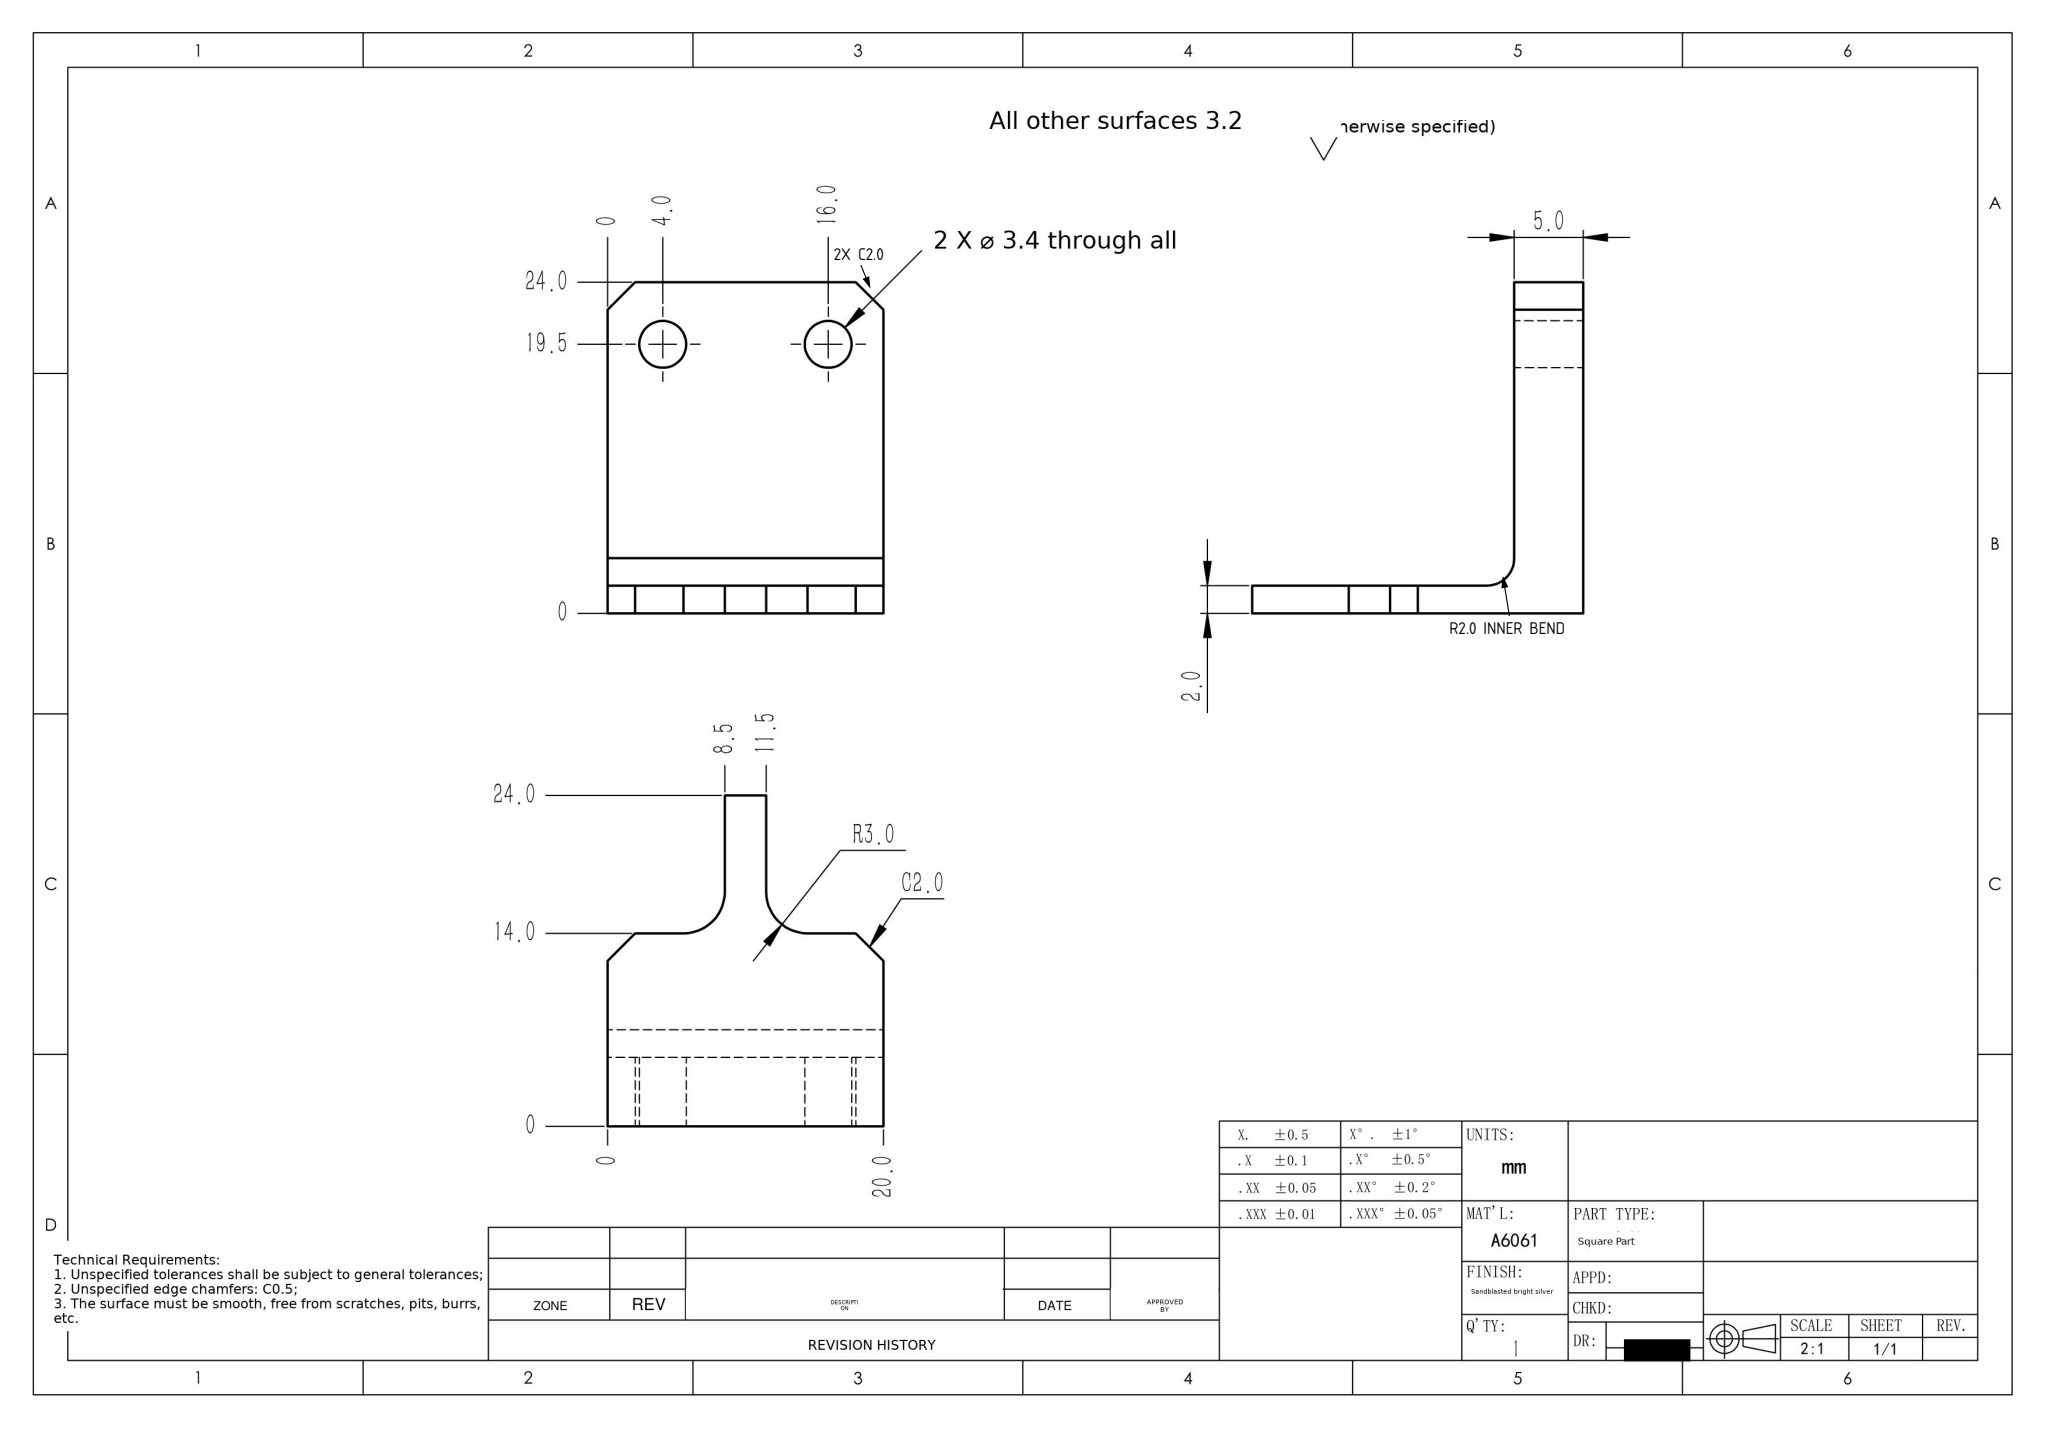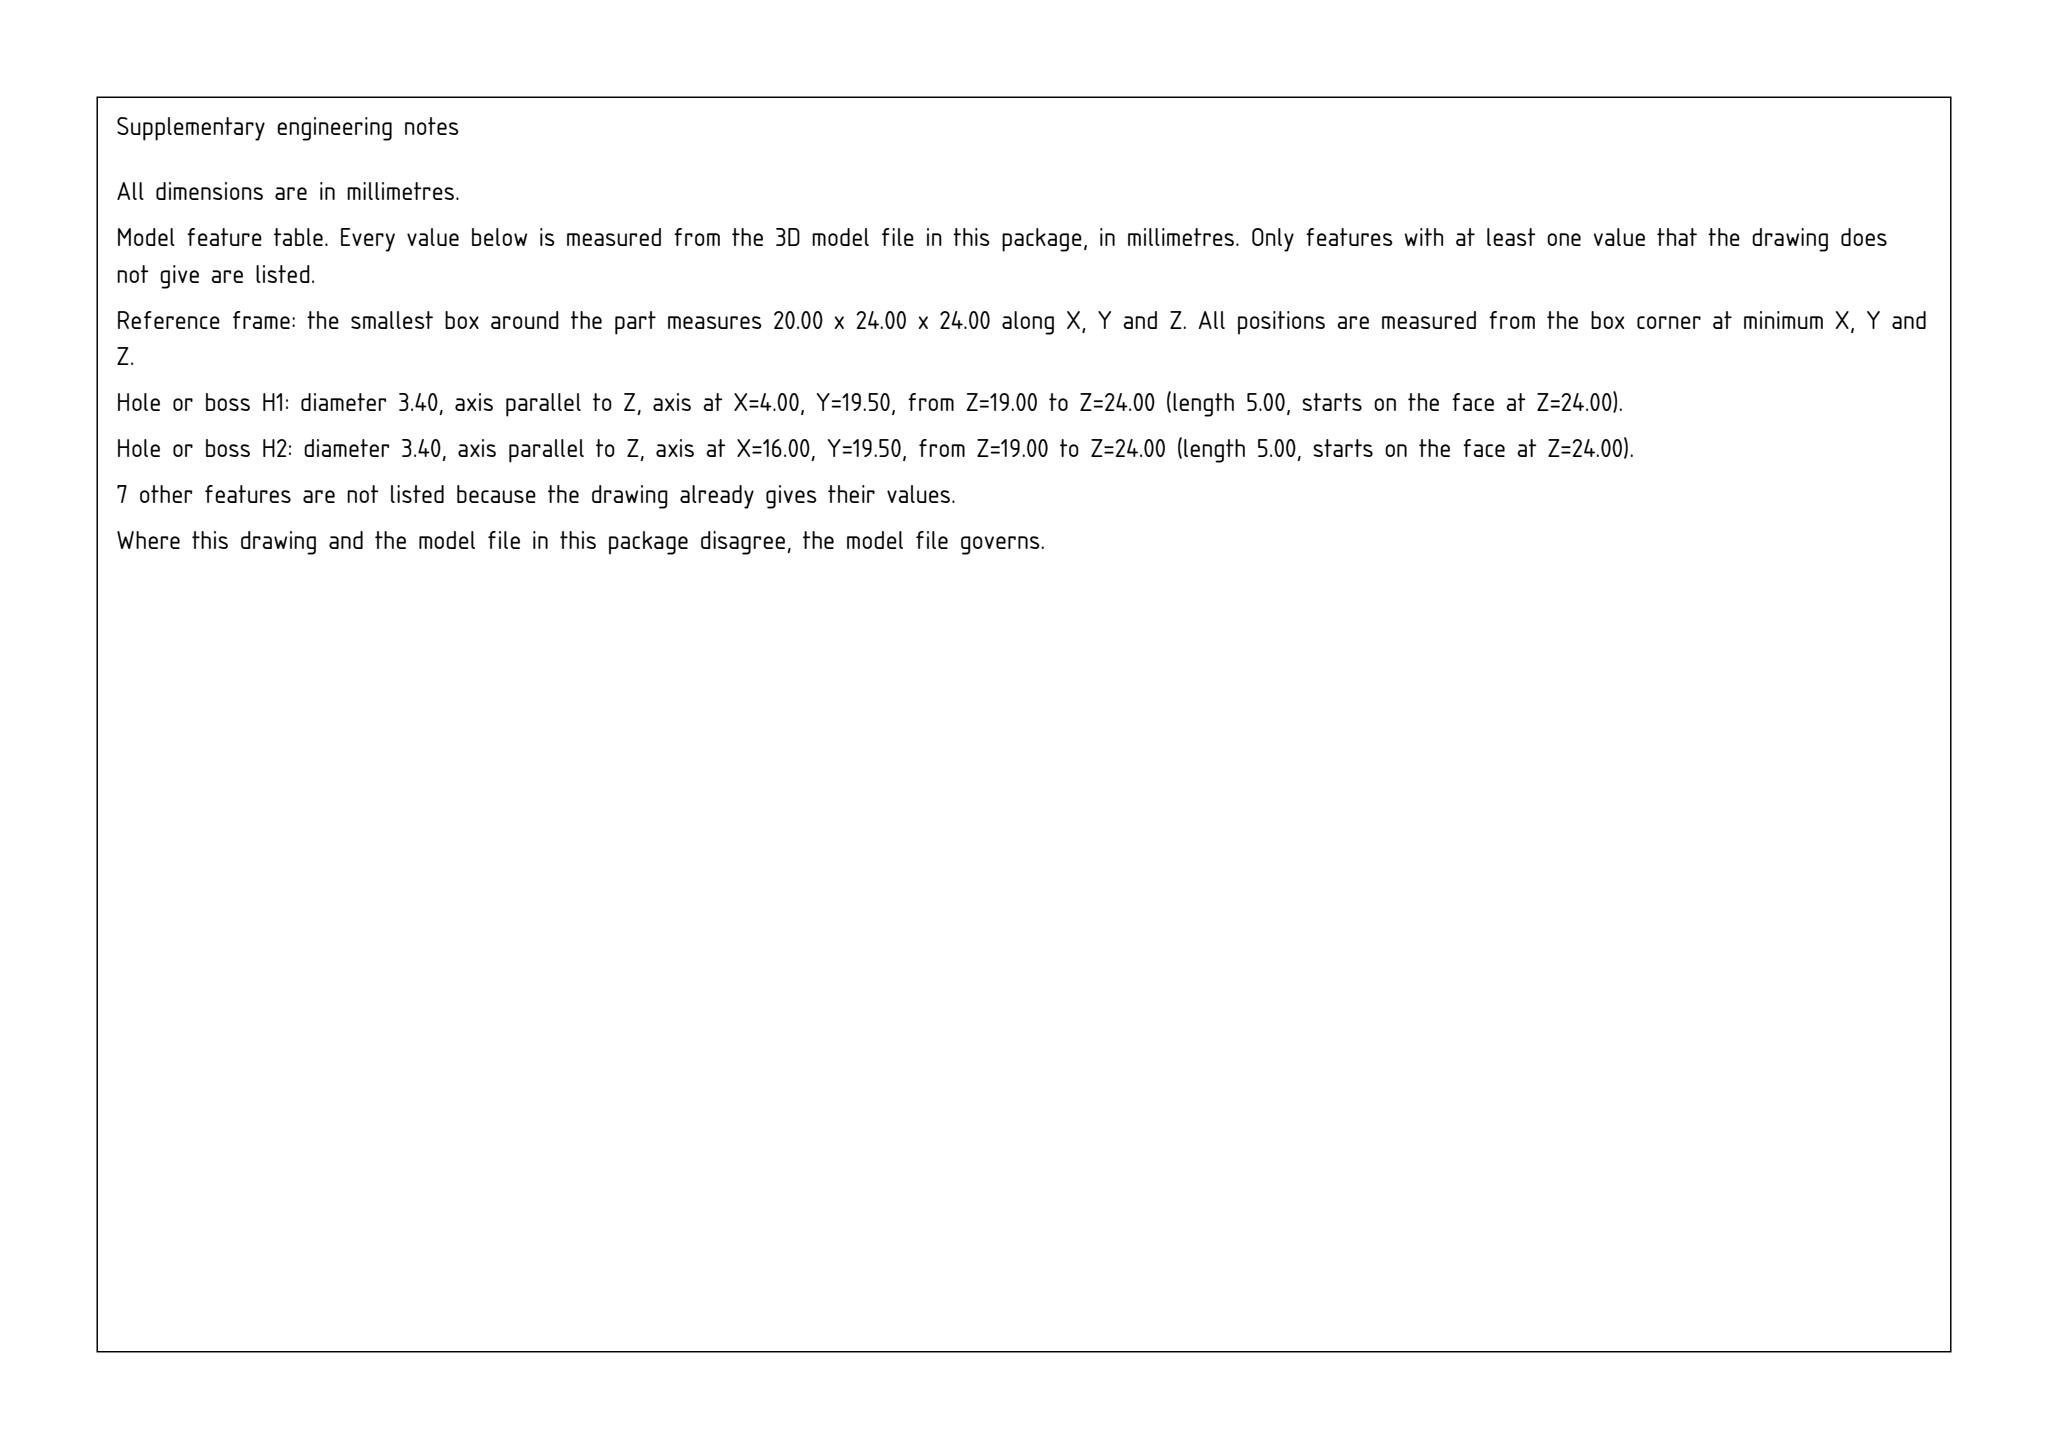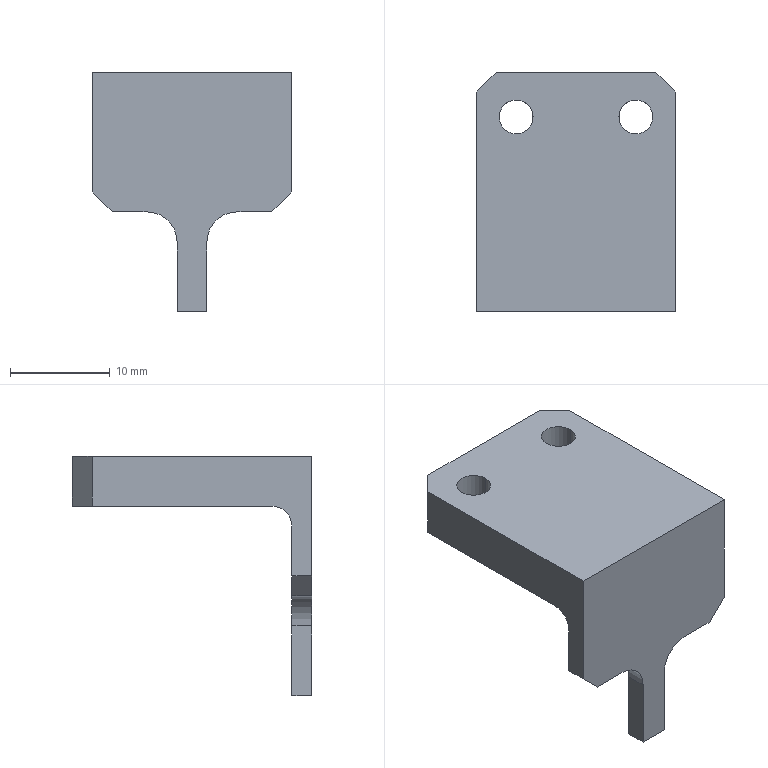Part | SolidWorks | mm | material A6061 | 1 solid | 23 faces | box 20 x 24 x 24 mm | volume 2726 mm3 | plane 16 | cylinder 7 | commonest cylinder face diameters 3.4 x4 6 x2 4 x1
Drawing notes:
INNER BEND FILLET R2.0 AT BASE-TO-UPRIGHT JUNCTION, FULL 20.0 WIDTH; ARC CENTER 4.0 FROM BOTTOM FACE (Y0) AND 17.0 FROM Z0 DATUM FACE. | from the solid: cylinders: [4.0 dia, axis x, pos y=4.0 z=17.0, length 20.0] -> R2.0 internal fillet tangent to base top face (y=2.0 plane) and upright inner face (z=19.0 plane)
2X CHAMFER 2.0 X 45° ON TOP CORNERS OF UPRIGHT: AT X=0 AND X=18 (20.0 WIDTH EDGES), RUNNING FROM Y=22.0 UP TO THE Y=24.0 TOP FACE, FULL 5.0 UPRIGHT THICKNESS (Z=19.0 TO 24.0 FROM MIN-CORNER DATUM) | from the solid: inclined_planes: angle_to_xyz_axes [45.0,45.0,90.0], bbox_from [0.0,22.0,19.0] size [2.0,2.0,5.0]; and bbox_from [18.0,22.0,19.0] size [2.0,2.0,5.0]
build123d program:
from build123d import *

# Parameters (mm, degrees)
SKETCH1_W            = 20
SKETCH1_H            = 24
BOSS_EXTRUDE1_DEPTH  = 24
SKETCH2_W            = 20
SKETCH2_H            = 22
CUT_EXTRUDE1_DEPTH   = 19
SKETCH3_W            = 8.5
SKETCH3_H            = 2
CUT_EXTRUDE2_DEPTH   = 10
M3_CLEARANCE_HOLE1_D = 3.4
CHAMFER1_SIZE        = 2
FILLET1_R            = 3
FILLET2_R            = 2


with BuildPart() as part:
    # Sketch1 → Boss-Extrude1 (new body)
    with BuildSketch(Plane.XY):
        with Locations((0, -12)):
            Rectangle(SKETCH1_W, SKETCH1_H)
    extrude(amount=BOSS_EXTRUDE1_DEPTH)

    # Sketch2 → Cut-Extrude1 (cut)
    with BuildSketch(Plane(origin=(0, 0, 0), x_dir=(-1, 0, 0), z_dir=(0, 0, -1))):
        with Locations((0, -11)):
            Rectangle(SKETCH2_W, SKETCH2_H)
    extrude(amount=-CUT_EXTRUDE1_DEPTH, mode=Mode.SUBTRACT)

    # Sketch3 → Cut-Extrude2 (cut)
    with BuildSketch(Plane(origin=(0, 0, 0), x_dir=(-1, 0, 0), z_dir=(0, 0, -1))):
        with Locations((-5.75, -23)):
            Rectangle(SKETCH3_W, SKETCH3_H)
        with Locations((5.75, -23)):
            Rectangle(SKETCH3_W, SKETCH3_H)
    extrude(amount=-CUT_EXTRUDE2_DEPTH, mode=Mode.SUBTRACT)

    # M3 Clearance Hole1 (through all)
    with Locations(Plane.XY.offset(24)):
        with Locations((-6, -4.5), (6, -4.5)):
            Hole(M3_CLEARANCE_HOLE1_D / 2)

    # Chamfer1
    chamfer1_edges = [part.edges().sort_by_distance(p)[0] for p in [
        (10, -23, 10),
        (-10, -23, 10),
        (-10, 0, 21.5),
        (10, 0, 21.5),
    ]]
    chamfer(chamfer1_edges, length=CHAMFER1_SIZE)

    # Fillet1
    fillet1_edges = [part.edges().sort_by_distance(p)[0] for p in [
        (1.5, -23, 10),
        (-1.5, -23, 10),
    ]]
    fillet(fillet1_edges, radius=FILLET1_R)

    # Fillet2
    fillet2_edges = [part.edges().sort_by_distance(p)[0] for p in [
        (0, -22, 19),
    ]]
    fillet(fillet2_edges, radius=FILLET2_R)


solid = part.part
STEP:
#1=CARTESIAN_POINT('',(-7.7,-4.5,19.));
#2=VERTEX_POINT('',#1);
#3=CARTESIAN_POINT('',(-4.3,-4.5,19.));
#4=VERTEX_POINT('',#3);
#5=CARTESIAN_POINT('',(-6.,-4.5,19.));
#6=DIRECTION('',(0.,0.,1.));
#7=DIRECTION('',(1.,0.,0.));
#8=AXIS2_PLACEMENT_3D('',#5,#6,#7);
#9=CIRCLE('',#8,1.7);
#10=EDGE_CURVE('',#2,#4,#9,.T.);
#11=ORIENTED_EDGE('',*,*,#10,.F.);
#12=CARTESIAN_POINT('',(-7.7,-4.5,24.));
#13=VERTEX_POINT('',#12);
#14=CARTESIAN_POINT('',(-7.7,-4.5,24.));
#15=DIRECTION('',(0.,0.,1.));
#16=VECTOR('',#15,1000.);
#17=LINE('',#14,#16);
#18=EDGE_CURVE('',#2,#13,#17,.T.);
#19=ORIENTED_EDGE('',*,*,#18,.T.);
#20=CARTESIAN_POINT('',(-4.3,-4.5,24.));
#21=VERTEX_POINT('',#20);
#22=CARTESIAN_POINT('',(-6.,-4.5,24.));
#23=DIRECTION('',(0.,0.,1.));
#24=DIRECTION('',(1.,0.,0.));
#25=AXIS2_PLACEMENT_3D('',#22,#23,#24);
#26=CIRCLE('',#25,1.7);
#27=EDGE_CURVE('',#13,#21,#26,.T.);
#28=ORIENTED_EDGE('',*,*,#27,.T.);
#29=CARTESIAN_POINT('',(-4.3,-4.5,24.));
#30=DIRECTION('',(0.,0.,1.));
#31=VECTOR('',#30,1000.);
#32=LINE('',#29,#31);
#33=EDGE_CURVE('',#4,#21,#32,.T.);
#34=ORIENTED_EDGE('',*,*,#33,.F.);
#35=EDGE_LOOP('',(#11,#19,#28,#34));
#36=FACE_OUTER_BOUND('',#35,.T.);
#37=CARTESIAN_POINT('',(-6.,-4.5,24.));
#38=DIRECTION('',(0.,0.,1.));
#39=DIRECTION('',(1.,0.,0.));
#40=AXIS2_PLACEMENT_3D('',#37,#38,#39);
#41=CYLINDRICAL_SURFACE('',#40,1.7);
#42=ADVANCED_FACE('',(#36),#41,.F.);
#43=CARTESIAN_POINT('',(4.3,-4.5,19.));
#44=VERTEX_POINT('',#43);
#45=CARTESIAN_POINT('',(7.7,-4.5,19.));
#46=VERTEX_POINT('',#45);
#47=CARTESIAN_POINT('',(6.,-4.5,19.));
#48=DIRECTION('',(0.,0.,1.));
#49=DIRECTION('',(1.,0.,0.));
#50=AXIS2_PLACEMENT_3D('',#47,#48,#49);
#51=CIRCLE('',#50,1.7);
#52=EDGE_CURVE('',#44,#46,#51,.T.);
#53=ORIENTED_EDGE('',*,*,#52,.F.);
#54=CARTESIAN_POINT('',(4.3,-4.5,24.));
#55=VERTEX_POINT('',#54);
#56=CARTESIAN_POINT('',(4.3,-4.5,24.));
#57=DIRECTION('',(0.,0.,1.));
#58=VECTOR('',#57,1000.);
#59=LINE('',#56,#58);
#60=EDGE_CURVE('',#44,#55,#59,.T.);
#61=ORIENTED_EDGE('',*,*,#60,.T.);
#62=CARTESIAN_POINT('',(7.7,-4.5,24.));
#63=VERTEX_POINT('',#62);
#64=CARTESIAN_POINT('',(6.,-4.5,24.));
#65=DIRECTION('',(0.,0.,1.));
#66=DIRECTION('',(1.,0.,0.));
#67=AXIS2_PLACEMENT_3D('',#64,#65,#66);
#68=CIRCLE('',#67,1.7);
#69=EDGE_CURVE('',#55,#63,#68,.T.);
#70=ORIENTED_EDGE('',*,*,#69,.T.);
#71=CARTESIAN_POINT('',(7.7,-4.5,24.));
#72=DIRECTION('',(0.,0.,1.));
#73=VECTOR('',#72,1000.);
#74=LINE('',#71,#73);
#75=EDGE_CURVE('',#46,#63,#74,.T.);
#76=ORIENTED_EDGE('',*,*,#75,.F.);
#77=EDGE_LOOP('',(#53,#61,#70,#76));
#78=FACE_OUTER_BOUND('',#77,.T.);
#79=CARTESIAN_POINT('',(6.,-4.5,24.));
#80=DIRECTION('',(0.,0.,1.));
#81=DIRECTION('',(1.,0.,0.));
#82=AXIS2_PLACEMENT_3D('',#79,#80,#81);
#83=CYLINDRICAL_SURFACE('',#82,1.7);
#84=ADVANCED_FACE('',(#78),#83,.F.);
#85=CARTESIAN_POINT('',(-10.,-20.,19.));
#86=VERTEX_POINT('',#85);
#87=CARTESIAN_POINT('',(-10.,-2.,19.));
#88=VERTEX_POINT('',#87);
#89=CARTESIAN_POINT('',(-10.,0.,19.));
#90=DIRECTION('',(0.,1.,0.));
#91=VECTOR('',#90,1000.);
#92=LINE('',#89,#91);
#93=EDGE_CURVE('',#86,#88,#92,.T.);
#94=ORIENTED_EDGE('',*,*,#93,.F.);
#95=CARTESIAN_POINT('',(-10.,-22.,17.));
#96=VERTEX_POINT('',#95);
#97=CARTESIAN_POINT('',(-10.,-20.,17.));
#98=DIRECTION('',(1.,0.,0.));
#99=DIRECTION('',(0.,1.,0.));
#100=AXIS2_PLACEMENT_3D('',#97,#98,#99);
#101=CIRCLE('',#100,2.);
#102=EDGE_CURVE('',#86,#96,#101,.T.);
#103=ORIENTED_EDGE('',*,*,#102,.T.);
#104=CARTESIAN_POINT('',(-10.,-22.,12.));
#105=VERTEX_POINT('',#104);
#106=CARTESIAN_POINT('',(-10.,-22.,53.732));
#107=DIRECTION('',(0.,0.,-1.));
#108=VECTOR('',#107,1000.);
#109=LINE('',#106,#108);
#110=EDGE_CURVE('',#96,#105,#109,.T.);
#111=ORIENTED_EDGE('',*,*,#110,.T.);
#112=CARTESIAN_POINT('',(-10.,-24.,12.));
#113=VERTEX_POINT('',#112);
#114=CARTESIAN_POINT('',(-10.,-24.,12.));
#115=DIRECTION('',(0.,-1.,0.));
#116=VECTOR('',#115,1000.);
#117=LINE('',#114,#116);
#118=EDGE_CURVE('',#105,#113,#117,.T.);
#119=ORIENTED_EDGE('',*,*,#118,.T.);
#120=CARTESIAN_POINT('',(-10.,-24.,24.));
#121=VERTEX_POINT('',#120);
#122=CARTESIAN_POINT('',(-10.,-24.,24.));
#123=DIRECTION('',(0.,0.,-1.));
#124=VECTOR('',#123,1000.);
#125=LINE('',#122,#124);
#126=EDGE_CURVE('',#121,#113,#125,.T.);
#127=ORIENTED_EDGE('',*,*,#126,.F.);
#128=CARTESIAN_POINT('',(-10.,-2.,24.));
#129=VERTEX_POINT('',#128);
#130=CARTESIAN_POINT('',(-10.,0.,24.));
#131=DIRECTION('',(0.,-1.,0.));
#132=VECTOR('',#131,1000.);
#133=LINE('',#130,#132);
#134=EDGE_CURVE('',#129,#121,#133,.T.);
#135=ORIENTED_EDGE('',*,*,#134,.F.);
#136=CARTESIAN_POINT('',(-10.,-2.,24.));
#137=DIRECTION('',(0.,0.,-1.));
#138=VECTOR('',#137,1000.);
#139=LINE('',#136,#138);
#140=EDGE_CURVE('',#129,#88,#139,.T.);
#141=ORIENTED_EDGE('',*,*,#140,.T.);
#142=EDGE_LOOP('',(#94,#103,#111,#119,#127,#135,#141));
#143=FACE_OUTER_BOUND('',#142,.T.);
#144=CARTESIAN_POINT('',(-10.,0.,24.));
#145=DIRECTION('',(1.,0.,0.));
#146=DIRECTION('',(-0.,1.,0.));
#147=AXIS2_PLACEMENT_3D('',#144,#145,#146);
#148=PLANE('',#147);
#149=ADVANCED_FACE('',(#143),#148,.F.);
#150=CARTESIAN_POINT('',(10.,-24.,24.));
#151=VERTEX_POINT('',#150);
#152=CARTESIAN_POINT('',(10.,-24.,12.));
#153=VERTEX_POINT('',#152);
#154=CARTESIAN_POINT('',(10.,-24.,24.));
#155=DIRECTION('',(0.,0.,-1.));
#156=VECTOR('',#155,1000.);
#157=LINE('',#154,#156);
#158=EDGE_CURVE('',#151,#153,#157,.T.);
#159=ORIENTED_EDGE('',*,*,#158,.T.);
#160=CARTESIAN_POINT('',(10.,-22.,12.));
#161=VERTEX_POINT('',#160);
#162=CARTESIAN_POINT('',(10.,-22.,12.));
#163=DIRECTION('',(0.,1.,0.));
#164=VECTOR('',#163,1000.);
#165=LINE('',#162,#164);
#166=EDGE_CURVE('',#153,#161,#165,.T.);
#167=ORIENTED_EDGE('',*,*,#166,.T.);
#168=CARTESIAN_POINT('',(10.,-22.,17.));
#169=VERTEX_POINT('',#168);
#170=CARTESIAN_POINT('',(10.,-22.,53.732));
#171=DIRECTION('',(0.,0.,-1.));
#172=VECTOR('',#171,1000.);
#173=LINE('',#170,#172);
#174=EDGE_CURVE('',#169,#161,#173,.T.);
#175=ORIENTED_EDGE('',*,*,#174,.F.);
#176=CARTESIAN_POINT('',(10.,-20.,19.));
#177=VERTEX_POINT('',#176);
#178=CARTESIAN_POINT('',(10.,-20.,17.));
#179=DIRECTION('',(-1.,0.,0.));
#180=DIRECTION('',(0.,-1.,0.));
#181=AXIS2_PLACEMENT_3D('',#178,#179,#180);
#182=CIRCLE('',#181,2.);
#183=EDGE_CURVE('',#169,#177,#182,.T.);
#184=ORIENTED_EDGE('',*,*,#183,.T.);
#185=CARTESIAN_POINT('',(10.,-2.,19.));
#186=VERTEX_POINT('',#185);
#187=CARTESIAN_POINT('',(10.,0.,19.));
#188=DIRECTION('',(-0.,-1.,0.));
#189=VECTOR('',#188,1000.);
#190=LINE('',#187,#189);
#191=EDGE_CURVE('',#186,#177,#190,.T.);
#192=ORIENTED_EDGE('',*,*,#191,.F.);
#193=CARTESIAN_POINT('',(10.,-2.,24.));
#194=VERTEX_POINT('',#193);
#195=CARTESIAN_POINT('',(10.,-2.,24.));
#196=DIRECTION('',(0.,0.,1.));
#197=VECTOR('',#196,1000.);
#198=LINE('',#195,#197);
#199=EDGE_CURVE('',#186,#194,#198,.T.);
#200=ORIENTED_EDGE('',*,*,#199,.T.);
#201=CARTESIAN_POINT('',(10.,0.,24.));
#202=DIRECTION('',(0.,1.,0.));
#203=VECTOR('',#202,1000.);
#204=LINE('',#201,#203);
#205=EDGE_CURVE('',#151,#194,#204,.T.);
#206=ORIENTED_EDGE('',*,*,#205,.F.);
#207=EDGE_LOOP('',(#159,#167,#175,#184,#192,#200,#206));
#208=FACE_OUTER_BOUND('',#207,.T.);
#209=CARTESIAN_POINT('',(10.,0.,24.));
#210=DIRECTION('',(-1.,0.,0.));
#211=DIRECTION('',(-0.,-1.,0.));
#212=AXIS2_PLACEMENT_3D('',#209,#210,#211);
#213=PLANE('',#212);
#214=ADVANCED_FACE('',(#208),#213,.F.);
#215=CARTESIAN_POINT('',(8.,-24.,10.));
#216=VERTEX_POINT('',#215);
#217=CARTESIAN_POINT('',(4.5,-24.,10.));
#218=VERTEX_POINT('',#217);
#219=CARTESIAN_POINT('',(10.,-24.,10.));
#220=DIRECTION('',(-1.,0.,0.));
#221=VECTOR('',#220,1000.);
#222=LINE('',#219,#221);
#223=EDGE_CURVE('',#216,#218,#222,.T.);
#224=ORIENTED_EDGE('',*,*,#223,.F.);
#225=CARTESIAN_POINT('',(8.,-24.,10.));
#226=DIRECTION('',(0.7071,0.,0.7071));
#227=VECTOR('',#226,1000.);
#228=LINE('',#225,#227);
#229=EDGE_CURVE('',#216,#153,#228,.T.);
#230=ORIENTED_EDGE('',*,*,#229,.T.);
#231=ORIENTED_EDGE('',*,*,#158,.F.);
#232=CARTESIAN_POINT('',(-10.,-24.,24.));
#233=DIRECTION('',(1.,0.,0.));
#234=VECTOR('',#233,1000.);
#235=LINE('',#232,#234);
#236=EDGE_CURVE('',#121,#151,#235,.T.);
#237=ORIENTED_EDGE('',*,*,#236,.F.);
#238=ORIENTED_EDGE('',*,*,#126,.T.);
#239=CARTESIAN_POINT('',(-8.,-24.,10.));
#240=VERTEX_POINT('',#239);
#241=CARTESIAN_POINT('',(-8.,-24.,10.));
#242=DIRECTION('',(0.7071,0.,-0.7071));
#243=VECTOR('',#242,1000.);
#244=LINE('',#241,#243);
#245=EDGE_CURVE('',#113,#240,#244,.T.);
#246=ORIENTED_EDGE('',*,*,#245,.T.);
#247=CARTESIAN_POINT('',(-4.5,-24.,10.));
#248=VERTEX_POINT('',#247);
#249=CARTESIAN_POINT('',(-10.,-24.,10.));
#250=DIRECTION('',(-1.,0.,0.));
#251=VECTOR('',#250,1000.);
#252=LINE('',#249,#251);
#253=EDGE_CURVE('',#248,#240,#252,.T.);
#254=ORIENTED_EDGE('',*,*,#253,.F.);
#255=CARTESIAN_POINT('',(-1.5,-24.,7.));
#256=VERTEX_POINT('',#255);
#257=CARTESIAN_POINT('',(-4.5,-24.,7.));
#258=DIRECTION('',(0.,1.,0.));
#259=DIRECTION('',(0.,0.,1.));
#260=AXIS2_PLACEMENT_3D('',#257,#258,#259);
#261=CIRCLE('',#260,3.);
#262=EDGE_CURVE('',#248,#256,#261,.T.);
#263=ORIENTED_EDGE('',*,*,#262,.T.);
#264=CARTESIAN_POINT('',(-1.5,-24.,0.));
#265=VERTEX_POINT('',#264);
#266=CARTESIAN_POINT('',(-1.5,-24.,10.));
#267=DIRECTION('',(0.,0.,-1.));
#268=VECTOR('',#267,1000.);
#269=LINE('',#266,#268);
#270=EDGE_CURVE('',#256,#265,#269,.T.);
#271=ORIENTED_EDGE('',*,*,#270,.T.);
#272=CARTESIAN_POINT('',(1.5,-24.,0.));
#273=VERTEX_POINT('',#272);
#274=CARTESIAN_POINT('',(-10.,-24.,0.));
#275=DIRECTION('',(1.,0.,0.));
#276=VECTOR('',#275,1000.);
#277=LINE('',#274,#276);
#278=EDGE_CURVE('',#265,#273,#277,.T.);
#279=ORIENTED_EDGE('',*,*,#278,.T.);
#280=CARTESIAN_POINT('',(1.5,-24.,7.));
#281=VERTEX_POINT('',#280);
#282=CARTESIAN_POINT('',(1.5,-24.,10.));
#283=DIRECTION('',(0.,0.,-1.));
#284=VECTOR('',#283,1000.);
#285=LINE('',#282,#284);
#286=EDGE_CURVE('',#281,#273,#285,.T.);
#287=ORIENTED_EDGE('',*,*,#286,.F.);
#288=CARTESIAN_POINT('',(4.5,-24.,7.));
#289=DIRECTION('',(0.,1.,0.));
#290=DIRECTION('',(0.,0.,1.));
#291=AXIS2_PLACEMENT_3D('',#288,#289,#290);
#292=CIRCLE('',#291,3.);
#293=EDGE_CURVE('',#281,#218,#292,.T.);
#294=ORIENTED_EDGE('',*,*,#293,.T.);
#295=EDGE_LOOP('',(#224,#230,#231,#237,#238,#246,#254,#263,#271,#279,#287,#294));
#296=FACE_OUTER_BOUND('',#295,.T.);
#297=CARTESIAN_POINT('',(-10.,-24.,24.));
#298=DIRECTION('',(0.,1.,0.));
#299=DIRECTION('',(0.,0.,1.));
#300=AXIS2_PLACEMENT_3D('',#297,#298,#299);
#301=PLANE('',#300);
#302=ADVANCED_FACE('',(#296),#301,.F.);
#303=CARTESIAN_POINT('',(-8.,0.,19.));
#304=VERTEX_POINT('',#303);
#305=CARTESIAN_POINT('',(8.,0.,19.));
#306=VERTEX_POINT('',#305);
#307=CARTESIAN_POINT('',(10.,0.,19.));
#308=DIRECTION('',(1.,0.,0.));
#309=VECTOR('',#308,1000.);
#310=LINE('',#307,#309);
#311=EDGE_CURVE('',#304,#306,#310,.T.);
#312=ORIENTED_EDGE('',*,*,#311,.F.);
#313=CARTESIAN_POINT('',(-8.,0.,24.));
#314=VERTEX_POINT('',#313);
#315=CARTESIAN_POINT('',(-8.,0.,24.));
#316=DIRECTION('',(0.,0.,1.));
#317=VECTOR('',#316,1000.);
#318=LINE('',#315,#317);
#319=EDGE_CURVE('',#304,#314,#318,.T.);
#320=ORIENTED_EDGE('',*,*,#319,.T.);
#321=CARTESIAN_POINT('',(8.,0.,24.));
#322=VERTEX_POINT('',#321);
#323=CARTESIAN_POINT('',(-10.,0.,24.));
#324=DIRECTION('',(-1.,0.,0.));
#325=VECTOR('',#324,1000.);
#326=LINE('',#323,#325);
#327=EDGE_CURVE('',#322,#314,#326,.T.);
#328=ORIENTED_EDGE('',*,*,#327,.F.);
#329=CARTESIAN_POINT('',(8.,0.,24.));
#330=DIRECTION('',(0.,0.,-1.));
#331=VECTOR('',#330,1000.);
#332=LINE('',#329,#331);
#333=EDGE_CURVE('',#322,#306,#332,.T.);
#334=ORIENTED_EDGE('',*,*,#333,.T.);
#335=EDGE_LOOP('',(#312,#320,#328,#334));
#336=FACE_OUTER_BOUND('',#335,.T.);
#337=CARTESIAN_POINT('',(-10.,0.,24.));
#338=DIRECTION('',(0.,-1.,0.));
#339=DIRECTION('',(0.,0.,-1.));
#340=AXIS2_PLACEMENT_3D('',#337,#338,#339);
#341=PLANE('',#340);
#342=ADVANCED_FACE('',(#336),#341,.F.);
#343=CARTESIAN_POINT('',(-6.,-4.5,24.));
#344=DIRECTION('',(0.,0.,1.));
#345=DIRECTION('',(1.,0.,0.));
#346=AXIS2_PLACEMENT_3D('',#343,#344,#345);
#347=CIRCLE('',#346,1.7);
#348=EDGE_CURVE('',#21,#13,#347,.T.);
#349=ORIENTED_EDGE('',*,*,#348,.F.);
#350=ORIENTED_EDGE('',*,*,#27,.F.);
#351=EDGE_LOOP('',(#349,#350));
#352=FACE_BOUND('',#351,.T.);
#353=CARTESIAN_POINT('',(6.,-4.5,24.));
#354=DIRECTION('',(0.,0.,1.));
#355=DIRECTION('',(1.,0.,0.));
#356=AXIS2_PLACEMENT_3D('',#353,#354,#355);
#357=CIRCLE('',#356,1.7);
#358=EDGE_CURVE('',#63,#55,#357,.T.);
#359=ORIENTED_EDGE('',*,*,#358,.F.);
#360=ORIENTED_EDGE('',*,*,#69,.F.);
#361=EDGE_LOOP('',(#359,#360));
#362=FACE_BOUND('',#361,.T.);
#363=ORIENTED_EDGE('',*,*,#327,.T.);
#364=CARTESIAN_POINT('',(-4.,4.,24.));
#365=DIRECTION('',(-0.7071,-0.7071,0.));
#366=VECTOR('',#365,1000.);
#367=LINE('',#364,#366);
#368=EDGE_CURVE('',#314,#129,#367,.T.);
#369=ORIENTED_EDGE('',*,*,#368,.T.);
#370=ORIENTED_EDGE('',*,*,#134,.T.);
#371=ORIENTED_EDGE('',*,*,#236,.T.);
#372=ORIENTED_EDGE('',*,*,#205,.T.);
#373=CARTESIAN_POINT('',(4.,4.,24.));
#374=DIRECTION('',(-0.7071,0.7071,0.));
#375=VECTOR('',#374,1000.);
#376=LINE('',#373,#375);
#377=EDGE_CURVE('',#194,#322,#376,.T.);
#378=ORIENTED_EDGE('',*,*,#377,.T.);
#379=EDGE_LOOP('',(#363,#369,#370,#371,#372,#378));
#380=FACE_OUTER_BOUND('',#379,.T.);
#381=CARTESIAN_POINT('',(0.,0.,24.));
#382=DIRECTION('',(0.,0.,1.));
#383=DIRECTION('',(1.,0.,0.));
#384=AXIS2_PLACEMENT_3D('',#381,#382,#383);
#385=PLANE('',#384);
#386=ADVANCED_FACE('',(#352,#362,#380),#385,.T.);
#387=ORIENTED_EDGE('',*,*,#278,.F.);
#388=CARTESIAN_POINT('',(-1.5,-22.,0.));
#389=VERTEX_POINT('',#388);
#390=CARTESIAN_POINT('',(-1.5,-22.,0.));
#391=DIRECTION('',(0.,-1.,0.));
#392=VECTOR('',#391,1000.);
#393=LINE('',#390,#392);
#394=EDGE_CURVE('',#389,#265,#393,.T.);
#395=ORIENTED_EDGE('',*,*,#394,.F.);
#396=CARTESIAN_POINT('',(1.5,-22.,0.));
#397=VERTEX_POINT('',#396);
#398=CARTESIAN_POINT('',(10.,-22.,0.));
#399=DIRECTION('',(-1.,0.,0.));
#400=VECTOR('',#399,1000.);
#401=LINE('',#398,#400);
#402=EDGE_CURVE('',#397,#389,#401,.T.);
#403=ORIENTED_EDGE('',*,*,#402,.F.);
#404=CARTESIAN_POINT('',(1.5,-22.,0.));
#405=DIRECTION('',(0.,1.,0.));
#406=VECTOR('',#405,1000.);
#407=LINE('',#404,#406);
#408=EDGE_CURVE('',#273,#397,#407,.T.);
#409=ORIENTED_EDGE('',*,*,#408,.F.);
#410=EDGE_LOOP('',(#387,#395,#403,#409));
#411=FACE_OUTER_BOUND('',#410,.T.);
#412=CARTESIAN_POINT('',(0.,0.,0.));
#413=DIRECTION('',(0.,0.,1.));
#414=DIRECTION('',(1.,0.,0.));
#415=AXIS2_PLACEMENT_3D('',#412,#413,#414);
#416=PLANE('',#415);
#417=ADVANCED_FACE('',(#411),#416,.F.);
#418=CARTESIAN_POINT('',(-6.,-4.5,19.));
#419=DIRECTION('',(0.,0.,1.));
#420=DIRECTION('',(1.,0.,0.));
#421=AXIS2_PLACEMENT_3D('',#418,#419,#420);
#422=CIRCLE('',#421,1.7);
#423=EDGE_CURVE('',#4,#2,#422,.T.);
#424=ORIENTED_EDGE('',*,*,#423,.T.);
#425=ORIENTED_EDGE('',*,*,#10,.T.);
#426=EDGE_LOOP('',(#424,#425));
#427=FACE_BOUND('',#426,.T.);
#428=CARTESIAN_POINT('',(6.,-4.5,19.));
#429=DIRECTION('',(0.,0.,1.));
#430=DIRECTION('',(1.,0.,0.));
#431=AXIS2_PLACEMENT_3D('',#428,#429,#430);
#432=CIRCLE('',#431,1.7);
#433=EDGE_CURVE('',#46,#44,#432,.T.);
#434=ORIENTED_EDGE('',*,*,#433,.T.);
#435=ORIENTED_EDGE('',*,*,#52,.T.);
#436=EDGE_LOOP('',(#434,#435));
#437=FACE_BOUND('',#436,.T.);
#438=ORIENTED_EDGE('',*,*,#191,.T.);
#439=CARTESIAN_POINT('',(-10.,-20.,19.));
#440=DIRECTION('',(-1.,0.,0.));
#441=VECTOR('',#440,1000.);
#442=LINE('',#439,#441);
#443=EDGE_CURVE('',#177,#86,#442,.T.);
#444=ORIENTED_EDGE('',*,*,#443,.T.);
#445=ORIENTED_EDGE('',*,*,#93,.T.);
#446=CARTESIAN_POINT('',(-10.,-2.,19.));
#447=DIRECTION('',(0.7071,0.7071,0.));
#448=VECTOR('',#447,1000.);
#449=LINE('',#446,#448);
#450=EDGE_CURVE('',#88,#304,#449,.T.);
#451=ORIENTED_EDGE('',*,*,#450,.T.);
#452=ORIENTED_EDGE('',*,*,#311,.T.);
#453=CARTESIAN_POINT('',(8.,0.,19.));
#454=DIRECTION('',(0.7071,-0.7071,0.));
#455=VECTOR('',#454,1000.);
#456=LINE('',#453,#455);
#457=EDGE_CURVE('',#306,#186,#456,.T.);
#458=ORIENTED_EDGE('',*,*,#457,.T.);
#459=EDGE_LOOP('',(#438,#444,#445,#451,#452,#458));
#460=FACE_OUTER_BOUND('',#459,.T.);
#461=CARTESIAN_POINT('',(0.,0.,19.));
#462=DIRECTION('',(0.,0.,1.));
#463=DIRECTION('',(1.,0.,0.));
#464=AXIS2_PLACEMENT_3D('',#461,#462,#463);
#465=PLANE('',#464);
#466=ADVANCED_FACE('',(#427,#437,#460),#465,.F.);
#467=ORIENTED_EDGE('',*,*,#110,.F.);
#468=CARTESIAN_POINT('',(10.,-22.,17.));
#469=DIRECTION('',(1.,0.,0.));
#470=VECTOR('',#469,1000.);
#471=LINE('',#468,#470);
#472=EDGE_CURVE('',#96,#169,#471,.T.);
#473=ORIENTED_EDGE('',*,*,#472,.T.);
#474=ORIENTED_EDGE('',*,*,#174,.T.);
#475=CARTESIAN_POINT('',(8.,-22.,10.));
#476=VERTEX_POINT('',#475);
#477=CARTESIAN_POINT('',(8.,-22.,10.));
#478=DIRECTION('',(-0.7071,0.,-0.7071));
#479=VECTOR('',#478,1000.);
#480=LINE('',#477,#479);
#481=EDGE_CURVE('',#161,#476,#480,.T.);
#482=ORIENTED_EDGE('',*,*,#481,.T.);
#483=CARTESIAN_POINT('',(4.5,-22.,10.));
#484=VERTEX_POINT('',#483);
#485=CARTESIAN_POINT('',(10.,-22.,10.));
#486=DIRECTION('',(1.,0.,0.));
#487=VECTOR('',#486,1000.);
#488=LINE('',#485,#487);
#489=EDGE_CURVE('',#484,#476,#488,.T.);
#490=ORIENTED_EDGE('',*,*,#489,.F.);
#491=CARTESIAN_POINT('',(1.5,-22.,7.));
#492=VERTEX_POINT('',#491);
#493=CARTESIAN_POINT('',(4.5,-22.,7.));
#494=DIRECTION('',(0.,-1.,0.));
#495=DIRECTION('',(0.,0.,-1.));
#496=AXIS2_PLACEMENT_3D('',#493,#494,#495);
#497=CIRCLE('',#496,3.);
#498=EDGE_CURVE('',#484,#492,#497,.T.);
#499=ORIENTED_EDGE('',*,*,#498,.T.);
#500=CARTESIAN_POINT('',(1.5,-22.,10.));
#501=DIRECTION('',(0.,0.,-1.));
#502=VECTOR('',#501,1000.);
#503=LINE('',#500,#502);
#504=EDGE_CURVE('',#492,#397,#503,.T.);
#505=ORIENTED_EDGE('',*,*,#504,.T.);
#506=ORIENTED_EDGE('',*,*,#402,.T.);
#507=CARTESIAN_POINT('',(-1.5,-22.,7.));
#508=VERTEX_POINT('',#507);
#509=CARTESIAN_POINT('',(-1.5,-22.,10.));
#510=DIRECTION('',(0.,0.,-1.));
#511=VECTOR('',#510,1000.);
#512=LINE('',#509,#511);
#513=EDGE_CURVE('',#508,#389,#512,.T.);
#514=ORIENTED_EDGE('',*,*,#513,.F.);
#515=CARTESIAN_POINT('',(-4.5,-22.,10.));
#516=VERTEX_POINT('',#515);
#517=CARTESIAN_POINT('',(-4.5,-22.,7.));
#518=DIRECTION('',(0.,-1.,0.));
#519=DIRECTION('',(0.,0.,-1.));
#520=AXIS2_PLACEMENT_3D('',#517,#518,#519);
#521=CIRCLE('',#520,3.);
#522=EDGE_CURVE('',#508,#516,#521,.T.);
#523=ORIENTED_EDGE('',*,*,#522,.T.);
#524=CARTESIAN_POINT('',(-8.,-22.,10.));
#525=VERTEX_POINT('',#524);
#526=CARTESIAN_POINT('',(-10.,-22.,10.));
#527=DIRECTION('',(1.,0.,0.));
#528=VECTOR('',#527,1000.);
#529=LINE('',#526,#528);
#530=EDGE_CURVE('',#525,#516,#529,.T.);
#531=ORIENTED_EDGE('',*,*,#530,.F.);
#532=CARTESIAN_POINT('',(-8.,-22.,10.));
#533=DIRECTION('',(-0.7071,0.,0.7071));
#534=VECTOR('',#533,1000.);
#535=LINE('',#532,#534);
#536=EDGE_CURVE('',#525,#105,#535,.T.);
#537=ORIENTED_EDGE('',*,*,#536,.T.);
#538=EDGE_LOOP('',(#467,#473,#474,#482,#490,#499,#505,#506,#514,#523,#531,#537));
#539=FACE_OUTER_BOUND('',#538,.T.);
#540=CARTESIAN_POINT('',(10.,-22.,53.732));
#541=DIRECTION('',(0.,-1.,0.));
#542=DIRECTION('',(0.,0.,-1.));
#543=AXIS2_PLACEMENT_3D('',#540,#541,#542);
#544=PLANE('',#543);
#545=ADVANCED_FACE('',(#539),#544,.F.);
#546=ORIENTED_EDGE('',*,*,#504,.F.);
#547=CARTESIAN_POINT('',(1.5,-22.,7.));
#548=DIRECTION('',(-0.,-1.,0.));
#549=VECTOR('',#548,1000.);
#550=LINE('',#547,#549);
#551=EDGE_CURVE('',#492,#281,#550,.T.);
#552=ORIENTED_EDGE('',*,*,#551,.T.);
#553=ORIENTED_EDGE('',*,*,#286,.T.);
#554=ORIENTED_EDGE('',*,*,#408,.T.);
#555=EDGE_LOOP('',(#546,#552,#553,#554));
#556=FACE_OUTER_BOUND('',#555,.T.);
#557=CARTESIAN_POINT('',(1.5,-22.,10.));
#558=DIRECTION('',(-1.,0.,0.));
#559=DIRECTION('',(-0.,-1.,0.));
#560=AXIS2_PLACEMENT_3D('',#557,#558,#559);
#561=PLANE('',#560);
#562=ADVANCED_FACE('',(#556),#561,.F.);
#563=ORIENTED_EDGE('',*,*,#223,.T.);
#564=CARTESIAN_POINT('',(4.5,-0.,10.));
#565=DIRECTION('',(0.,1.,0.));
#566=VECTOR('',#565,1000.);
#567=LINE('',#564,#566);
#568=EDGE_CURVE('',#218,#484,#567,.T.);
#569=ORIENTED_EDGE('',*,*,#568,.T.);
#570=ORIENTED_EDGE('',*,*,#489,.T.);
#571=CARTESIAN_POINT('',(8.,-24.,10.));
#572=DIRECTION('',(-0.,-1.,0.));
#573=VECTOR('',#572,1000.);
#574=LINE('',#571,#573);
#575=EDGE_CURVE('',#476,#216,#574,.T.);
#576=ORIENTED_EDGE('',*,*,#575,.T.);
#577=EDGE_LOOP('',(#563,#569,#570,#576));
#578=FACE_OUTER_BOUND('',#577,.T.);
#579=CARTESIAN_POINT('',(0.,0.,10.));
#580=DIRECTION('',(0.,0.,-1.));
#581=DIRECTION('',(-1.,0.,0.));
#582=AXIS2_PLACEMENT_3D('',#579,#580,#581);
#583=PLANE('',#582);
#584=ADVANCED_FACE('',(#578),#583,.T.);
#585=ORIENTED_EDGE('',*,*,#270,.F.);
#586=CARTESIAN_POINT('',(-1.5,-22.,7.));
#587=DIRECTION('',(-0.,1.,0.));
#588=VECTOR('',#587,1000.);
#589=LINE('',#586,#588);
#590=EDGE_CURVE('',#256,#508,#589,.T.);
#591=ORIENTED_EDGE('',*,*,#590,.T.);
#592=ORIENTED_EDGE('',*,*,#513,.T.);
#593=ORIENTED_EDGE('',*,*,#394,.T.);
#594=EDGE_LOOP('',(#585,#591,#592,#593));
#595=FACE_OUTER_BOUND('',#594,.T.);
#596=CARTESIAN_POINT('',(-1.5,-22.,10.));
#597=DIRECTION('',(1.,0.,0.));
#598=DIRECTION('',(-0.,1.,0.));
#599=AXIS2_PLACEMENT_3D('',#596,#597,#598);
#600=PLANE('',#599);
#601=ADVANCED_FACE('',(#595),#600,.F.);
#602=ORIENTED_EDGE('',*,*,#530,.T.);
#603=CARTESIAN_POINT('',(-4.5,-0.,10.));
#604=DIRECTION('',(0.,-1.,0.));
#605=VECTOR('',#604,1000.);
#606=LINE('',#603,#605);
#607=EDGE_CURVE('',#516,#248,#606,.T.);
#608=ORIENTED_EDGE('',*,*,#607,.T.);
#609=ORIENTED_EDGE('',*,*,#253,.T.);
#610=CARTESIAN_POINT('',(-8.,-22.,10.));
#611=DIRECTION('',(-0.,1.,0.));
#612=VECTOR('',#611,1000.);
#613=LINE('',#610,#612);
#614=EDGE_CURVE('',#240,#525,#613,.T.);
#615=ORIENTED_EDGE('',*,*,#614,.T.);
#616=EDGE_LOOP('',(#602,#608,#609,#615));
#617=FACE_OUTER_BOUND('',#616,.T.);
#618=CARTESIAN_POINT('',(0.,0.,10.));
#619=DIRECTION('',(0.,0.,-1.));
#620=DIRECTION('',(-1.,0.,0.));
#621=AXIS2_PLACEMENT_3D('',#618,#619,#620);
#622=PLANE('',#621);
#623=ADVANCED_FACE('',(#617),#622,.T.);
#624=ORIENTED_EDGE('',*,*,#60,.F.);
#625=ORIENTED_EDGE('',*,*,#433,.F.);
#626=ORIENTED_EDGE('',*,*,#75,.T.);
#627=ORIENTED_EDGE('',*,*,#358,.T.);
#628=EDGE_LOOP('',(#624,#625,#626,#627));
#629=FACE_OUTER_BOUND('',#628,.T.);
#630=CARTESIAN_POINT('',(6.,-4.5,24.));
#631=DIRECTION('',(0.,0.,1.));
#632=DIRECTION('',(1.,0.,0.));
#633=AXIS2_PLACEMENT_3D('',#630,#631,#632);
#634=CYLINDRICAL_SURFACE('',#633,1.7);
#635=ADVANCED_FACE('',(#629),#634,.F.);
#636=ORIENTED_EDGE('',*,*,#18,.F.);
#637=ORIENTED_EDGE('',*,*,#423,.F.);
#638=ORIENTED_EDGE('',*,*,#33,.T.);
#639=ORIENTED_EDGE('',*,*,#348,.T.);
#640=EDGE_LOOP('',(#636,#637,#638,#639));
#641=FACE_OUTER_BOUND('',#640,.T.);
#642=CARTESIAN_POINT('',(-6.,-4.5,24.));
#643=DIRECTION('',(0.,0.,1.));
#644=DIRECTION('',(1.,0.,0.));
#645=AXIS2_PLACEMENT_3D('',#642,#643,#644);
#646=CYLINDRICAL_SURFACE('',#645,1.7);
#647=ADVANCED_FACE('',(#641),#646,.F.);
#648=ORIENTED_EDGE('',*,*,#481,.F.);
#649=ORIENTED_EDGE('',*,*,#166,.F.);
#650=ORIENTED_EDGE('',*,*,#229,.F.);
#651=ORIENTED_EDGE('',*,*,#575,.F.);
#652=EDGE_LOOP('',(#648,#649,#650,#651));
#653=FACE_OUTER_BOUND('',#652,.T.);
#654=CARTESIAN_POINT('',(8.,-0.,10.));
#655=DIRECTION('',(0.7071,-0.,-0.7071));
#656=DIRECTION('',(0.,1.,0.));
#657=AXIS2_PLACEMENT_3D('',#654,#655,#656);
#658=PLANE('',#657);
#659=ADVANCED_FACE('',(#653),#658,.T.);
#660=ORIENTED_EDGE('',*,*,#245,.F.);
#661=ORIENTED_EDGE('',*,*,#118,.F.);
#662=ORIENTED_EDGE('',*,*,#536,.F.);
#663=ORIENTED_EDGE('',*,*,#614,.F.);
#664=EDGE_LOOP('',(#660,#661,#662,#663));
#665=FACE_OUTER_BOUND('',#664,.T.);
#666=CARTESIAN_POINT('',(-8.,-0.,10.));
#667=DIRECTION('',(-0.7071,-0.,-0.7071));
#668=DIRECTION('',(0.,-1.,0.));
#669=AXIS2_PLACEMENT_3D('',#666,#667,#668);
#670=PLANE('',#669);
#671=ADVANCED_FACE('',(#665),#670,.T.);
#672=ORIENTED_EDGE('',*,*,#368,.F.);
#673=ORIENTED_EDGE('',*,*,#319,.F.);
#674=ORIENTED_EDGE('',*,*,#450,.F.);
#675=ORIENTED_EDGE('',*,*,#140,.F.);
#676=EDGE_LOOP('',(#672,#673,#674,#675));
#677=FACE_OUTER_BOUND('',#676,.T.);
#678=CARTESIAN_POINT('',(-10.,-2.,24.));
#679=DIRECTION('',(0.7071,-0.7071,0.));
#680=DIRECTION('',(0.,0.,-1.));
#681=AXIS2_PLACEMENT_3D('',#678,#679,#680);
#682=PLANE('',#681);
#683=ADVANCED_FACE('',(#677),#682,.F.);
#684=ORIENTED_EDGE('',*,*,#377,.F.);
#685=ORIENTED_EDGE('',*,*,#199,.F.);
#686=ORIENTED_EDGE('',*,*,#457,.F.);
#687=ORIENTED_EDGE('',*,*,#333,.F.);
#688=EDGE_LOOP('',(#684,#685,#686,#687));
#689=FACE_OUTER_BOUND('',#688,.T.);
#690=CARTESIAN_POINT('',(8.,0.,24.));
#691=DIRECTION('',(-0.7071,-0.7071,0.));
#692=DIRECTION('',(0.,0.,-1.));
#693=AXIS2_PLACEMENT_3D('',#690,#691,#692);
#694=PLANE('',#693);
#695=ADVANCED_FACE('',(#689),#694,.F.);
#696=ORIENTED_EDGE('',*,*,#293,.F.);
#697=ORIENTED_EDGE('',*,*,#551,.F.);
#698=ORIENTED_EDGE('',*,*,#498,.F.);
#699=ORIENTED_EDGE('',*,*,#568,.F.);
#700=EDGE_LOOP('',(#696,#697,#698,#699));
#701=FACE_OUTER_BOUND('',#700,.T.);
#702=CARTESIAN_POINT('',(4.5,-0.,7.));
#703=DIRECTION('',(0.,1.,0.));
#704=DIRECTION('',(-1.,0.,0.));
#705=AXIS2_PLACEMENT_3D('',#702,#703,#704);
#706=CYLINDRICAL_SURFACE('',#705,3.);
#707=ADVANCED_FACE('',(#701),#706,.F.);
#708=ORIENTED_EDGE('',*,*,#522,.F.);
#709=ORIENTED_EDGE('',*,*,#590,.F.);
#710=ORIENTED_EDGE('',*,*,#262,.F.);
#711=ORIENTED_EDGE('',*,*,#607,.F.);
#712=EDGE_LOOP('',(#708,#709,#710,#711));
#713=FACE_OUTER_BOUND('',#712,.T.);
#714=CARTESIAN_POINT('',(-4.5,-0.,7.));
#715=DIRECTION('',(0.,-1.,0.));
#716=DIRECTION('',(1.,0.,0.));
#717=AXIS2_PLACEMENT_3D('',#714,#715,#716);
#718=CYLINDRICAL_SURFACE('',#717,3.);
#719=ADVANCED_FACE('',(#713),#718,.F.);
#720=ORIENTED_EDGE('',*,*,#183,.F.);
#721=ORIENTED_EDGE('',*,*,#472,.F.);
#722=ORIENTED_EDGE('',*,*,#102,.F.);
#723=ORIENTED_EDGE('',*,*,#443,.F.);
#724=EDGE_LOOP('',(#720,#721,#722,#723));
#725=FACE_OUTER_BOUND('',#724,.T.);
#726=CARTESIAN_POINT('',(0.,-20.,17.));
#727=DIRECTION('',(1.,0.,0.));
#728=DIRECTION('',(0.,0.,-1.));
#729=AXIS2_PLACEMENT_3D('',#726,#727,#728);
#730=CYLINDRICAL_SURFACE('',#729,2.);
#731=ADVANCED_FACE('',(#725),#730,.F.);
#732=CLOSED_SHELL('',(#42,#84,#149,#214,#302,#342,#386,#417,#466,#545,#562,#584,#601,#623,#635,#647,#659,#671,#683,#695,#707,#719,#731));
#733=MANIFOLD_SOLID_BREP('',#732);
#734=CARTESIAN_POINT('',(0.,0.,0.));
#735=DIRECTION('',(0.,0.,1.));
#736=DIRECTION('',(1.,0.,0.));
#737=AXIS2_PLACEMENT_3D('',#734,#735,#736);
#738=(LENGTH_UNIT()NAMED_UNIT(*)SI_UNIT(.MILLI.,.METRE.));
#739=UNCERTAINTY_MEASURE_WITH_UNIT(LENGTH_MEASURE(0.00001),#738,'','');
#740=(NAMED_UNIT(*)PLANE_ANGLE_UNIT()SI_UNIT($,.RADIAN.));
#741=(NAMED_UNIT(*)SI_UNIT($,.STERADIAN.)SOLID_ANGLE_UNIT());
#742=(GEOMETRIC_REPRESENTATION_CONTEXT(3)GLOBAL_UNCERTAINTY_ASSIGNED_CONTEXT((#739))GLOBAL_UNIT_ASSIGNED_CONTEXT((#738,#740,#741))REPRESENTATION_CONTEXT('',''));
#743=ADVANCED_BREP_SHAPE_REPRESENTATION('',(#733,#737),#742);